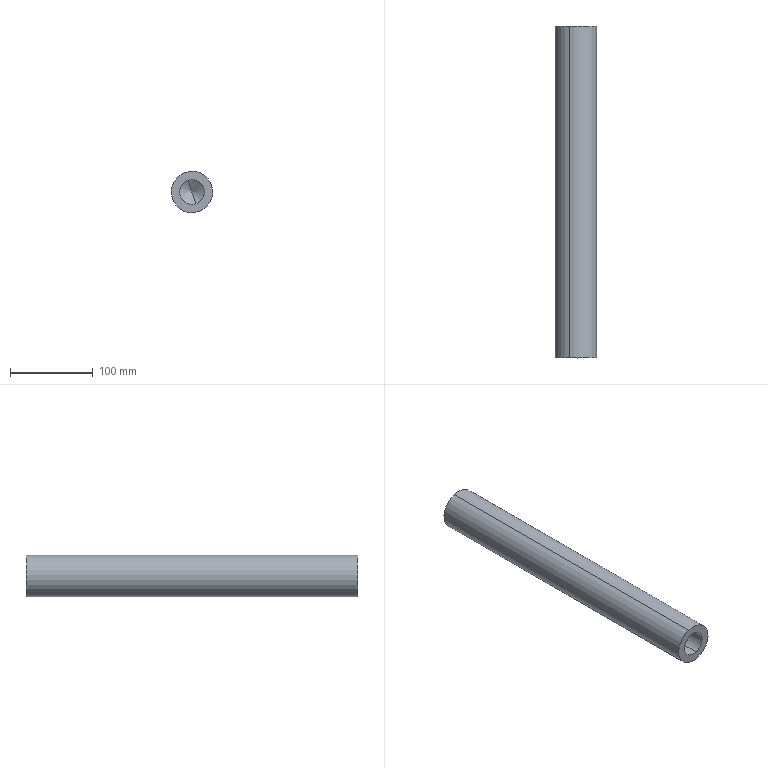Component | SolidWorks | AdjustingTieRod1-1 | 1 solid | 12 faces | box 50 x 400 x 50 mm | volume 639779 mm3 | cylinder 6 | cone 4 | plane 2 | commonest cylinder face diameters 30 x4 50 x2 | material N/A
build123d program:
from build123d import *

# Parameters (mm, degrees)
SKETCH2_R              = 25
BOSS_EXTRUDE1_DEPTH    = 400
M30_TAPPED_HOLE1_D     = 30
M30_TAPPED_HOLE1_DEPTH = 100
M30_TAPPED_HOLE1_TIP   = 9.013
M30_TAPPED_HOLE3_D     = 30
M30_TAPPED_HOLE3_DEPTH = 100
M30_TAPPED_HOLE3_TIP   = 9.013


with BuildPart() as part:
    # Sketch2 → Boss-Extrude1 (new body)
    with BuildSketch(Plane(origin=(0, 0, 0), x_dir=(1, 0, 0), z_dir=(0, 1, 0))):
        with Locations(Location((0, 0, 0), (0, 0, 270))):
            Circle(SKETCH2_R)
    extrude(amount=BOSS_EXTRUDE1_DEPTH)

    # M30 Tapped Hole1
    with Locations(Plane(origin=(0, 400, 0), x_dir=(1, 0, 0), z_dir=(0, 1, 0))):
        with Locations((0, 0)):
            Hole(M30_TAPPED_HOLE1_D / 2, depth=M30_TAPPED_HOLE1_DEPTH)
            with Locations((0, 0, -(M30_TAPPED_HOLE1_DEPTH + M30_TAPPED_HOLE1_TIP / 2))):  # 118° drill point
                Cone(0, M30_TAPPED_HOLE1_D / 2, M30_TAPPED_HOLE1_TIP, mode=Mode.SUBTRACT)

    # M30 Tapped Hole3
    with Locations(Plane(origin=(0, 0, 0), x_dir=(-1, 0, 0), z_dir=(0, -1, 0))):
        with Locations((0, 0)):
            Hole(M30_TAPPED_HOLE3_D / 2, depth=M30_TAPPED_HOLE3_DEPTH)
            with Locations((0, 0, -(M30_TAPPED_HOLE3_DEPTH + M30_TAPPED_HOLE3_TIP / 2))):  # 118° drill point
                Cone(0, M30_TAPPED_HOLE3_D / 2, M30_TAPPED_HOLE3_TIP, mode=Mode.SUBTRACT)


solid = part.part

# Placed as in the assembly
solid = solid.moved(Location((69.344, 357.787, 17), (0, 0, 0)))
STEP:
#1=COLOUR_RGB('',0.7922,0.8196,0.9333);
#2=FILL_AREA_STYLE_COLOUR('',#1);
#3=FILL_AREA_STYLE('',(#2));
#4=SURFACE_STYLE_FILL_AREA(#3);
#5=SURFACE_SIDE_STYLE('',(#4));
#6=SURFACE_STYLE_USAGE(.BOTH.,#5);
#7=PRESENTATION_STYLE_ASSIGNMENT((#6));
#8=CARTESIAN_POINT('',(2.547,18.023,1.231));
#9=VERTEX_POINT('',#8);
#10=CARTESIAN_POINT('',(2.913,18.023,0.1078));
#11=VERTEX_POINT('',#10);
#12=CARTESIAN_POINT('',(2.73,18.023,0.6693));
#13=DIRECTION('',(-0.,-1.,-0.));
#14=DIRECTION('',(0.3098,0.,-0.9508));
#15=AXIS2_PLACEMENT_3D('',#12,#13,#14);
#16=CIRCLE('',#15,0.5906);
#17=EDGE_CURVE('',#9,#11,#16,.T.);
#18=ORIENTED_EDGE('',*,*,#17,.F.);
#19=CARTESIAN_POINT('',(2.547,14.086,1.231));
#20=VERTEX_POINT('',#19);
#21=CARTESIAN_POINT('',(2.547,14.086,1.231));
#22=DIRECTION('',(-0.,-1.,-0.));
#23=VECTOR('',#22,39.37);
#24=LINE('',#21,#23);
#25=EDGE_CURVE('',#9,#20,#24,.T.);
#26=ORIENTED_EDGE('',*,*,#25,.T.);
#27=CARTESIAN_POINT('',(2.913,14.086,0.1078));
#28=VERTEX_POINT('',#27);
#29=CARTESIAN_POINT('',(2.73,14.086,0.6693));
#30=DIRECTION('',(-0.,-1.,-0.));
#31=DIRECTION('',(0.3098,0.,-0.9508));
#32=AXIS2_PLACEMENT_3D('',#29,#30,#31);
#33=CIRCLE('',#32,0.5906);
#34=EDGE_CURVE('',#20,#28,#33,.T.);
#35=ORIENTED_EDGE('',*,*,#34,.T.);
#36=CARTESIAN_POINT('',(2.913,14.086,0.1078));
#37=DIRECTION('',(-0.,-1.,-0.));
#38=VECTOR('',#37,39.37);
#39=LINE('',#36,#38);
#40=EDGE_CURVE('',#11,#28,#39,.T.);
#41=ORIENTED_EDGE('',*,*,#40,.F.);
#42=EDGE_LOOP('',(#18,#26,#35,#41));
#43=FACE_OUTER_BOUND('',#42,.T.);
#44=CARTESIAN_POINT('',(2.73,14.086,0.6693));
#45=DIRECTION('',(-0.,-1.,-0.));
#46=DIRECTION('',(0.3098,0.,-0.9508));
#47=AXIS2_PLACEMENT_3D('',#44,#45,#46);
#48=CYLINDRICAL_SURFACE('',#47,0.5906);
#49=ADVANCED_FACE('',(#43),#48,.F.);
#50=CARTESIAN_POINT('',(2.73,18.378,0.6693));
#51=VERTEX_POINT('',#50);
#52=CARTESIAN_POINT('',(2.913,18.023,0.1078));
#53=DIRECTION('',(0.2656,-0.515,-0.815));
#54=VECTOR('',#53,39.37);
#55=LINE('',#52,#54);
#56=EDGE_CURVE('',#51,#11,#55,.T.);
#57=ORIENTED_EDGE('',*,*,#56,.F.);
#58=CARTESIAN_POINT('',(2.547,18.023,1.231));
#59=DIRECTION('',(-0.2656,-0.515,0.815));
#60=VECTOR('',#59,39.37);
#61=LINE('',#58,#60);
#62=EDGE_CURVE('',#51,#9,#61,.T.);
#63=ORIENTED_EDGE('',*,*,#62,.T.);
#64=ORIENTED_EDGE('',*,*,#17,.T.);
#65=EDGE_LOOP('',(#57,#63,#64));
#66=FACE_OUTER_BOUND('',#65,.T.);
#67=CARTESIAN_POINT('',(2.73,18.023,0.6693));
#68=DIRECTION('',(-0.,-1.,-0.));
#69=DIRECTION('',(0.3098,0.,-0.9508));
#70=AXIS2_PLACEMENT_3D('',#67,#68,#69);
#71=CONICAL_SURFACE('',#70,0.5906,1.03);
#72=ADVANCED_FACE('',(#66),#71,.F.);
#73=CARTESIAN_POINT('',(2.913,25.897,0.1078));
#74=VERTEX_POINT('',#73);
#75=CARTESIAN_POINT('',(2.547,25.897,1.231));
#76=VERTEX_POINT('',#75);
#77=CARTESIAN_POINT('',(2.73,25.897,0.6693));
#78=DIRECTION('',(0.,1.,0.));
#79=DIRECTION('',(-0.3098,0.,0.9508));
#80=AXIS2_PLACEMENT_3D('',#77,#78,#79);
#81=CIRCLE('',#80,0.5906);
#82=EDGE_CURVE('',#74,#76,#81,.T.);
#83=ORIENTED_EDGE('',*,*,#82,.F.);
#84=CARTESIAN_POINT('',(2.913,29.834,0.1078));
#85=VERTEX_POINT('',#84);
#86=CARTESIAN_POINT('',(2.913,29.834,0.1078));
#87=DIRECTION('',(0.,1.,0.));
#88=VECTOR('',#87,39.37);
#89=LINE('',#86,#88);
#90=EDGE_CURVE('',#74,#85,#89,.T.);
#91=ORIENTED_EDGE('',*,*,#90,.T.);
#92=CARTESIAN_POINT('',(2.547,29.834,1.231));
#93=VERTEX_POINT('',#92);
#94=CARTESIAN_POINT('',(2.73,29.834,0.6693));
#95=DIRECTION('',(0.,1.,0.));
#96=DIRECTION('',(-0.3098,0.,0.9508));
#97=AXIS2_PLACEMENT_3D('',#94,#95,#96);
#98=CIRCLE('',#97,0.5906);
#99=EDGE_CURVE('',#85,#93,#98,.T.);
#100=ORIENTED_EDGE('',*,*,#99,.T.);
#101=CARTESIAN_POINT('',(2.547,29.834,1.231));
#102=DIRECTION('',(0.,1.,0.));
#103=VECTOR('',#102,39.37);
#104=LINE('',#101,#103);
#105=EDGE_CURVE('',#76,#93,#104,.T.);
#106=ORIENTED_EDGE('',*,*,#105,.F.);
#107=EDGE_LOOP('',(#83,#91,#100,#106));
#108=FACE_OUTER_BOUND('',#107,.T.);
#109=CARTESIAN_POINT('',(2.73,29.834,0.6693));
#110=DIRECTION('',(0.,1.,0.));
#111=DIRECTION('',(-0.3098,0.,0.9508));
#112=AXIS2_PLACEMENT_3D('',#109,#110,#111);
#113=CYLINDRICAL_SURFACE('',#112,0.5906);
#114=ADVANCED_FACE('',(#108),#113,.F.);
#115=CARTESIAN_POINT('',(2.73,25.542,0.6693));
#116=VERTEX_POINT('',#115);
#117=CARTESIAN_POINT('',(2.547,25.897,1.231));
#118=DIRECTION('',(-0.2656,0.515,0.815));
#119=VECTOR('',#118,39.37);
#120=LINE('',#117,#119);
#121=EDGE_CURVE('',#116,#76,#120,.T.);
#122=ORIENTED_EDGE('',*,*,#121,.F.);
#123=CARTESIAN_POINT('',(2.913,25.897,0.1078));
#124=DIRECTION('',(0.2656,0.515,-0.815));
#125=VECTOR('',#124,39.37);
#126=LINE('',#123,#125);
#127=EDGE_CURVE('',#116,#74,#126,.T.);
#128=ORIENTED_EDGE('',*,*,#127,.T.);
#129=ORIENTED_EDGE('',*,*,#82,.T.);
#130=EDGE_LOOP('',(#122,#128,#129));
#131=FACE_OUTER_BOUND('',#130,.T.);
#132=CARTESIAN_POINT('',(2.73,25.897,0.6693));
#133=DIRECTION('',(0.,1.,0.));
#134=DIRECTION('',(-0.3098,0.,0.9508));
#135=AXIS2_PLACEMENT_3D('',#132,#133,#134);
#136=CONICAL_SURFACE('',#135,0.5906,1.03);
#137=ADVANCED_FACE('',(#131),#136,.F.);
#138=CARTESIAN_POINT('',(2.425,29.834,1.605));
#139=VERTEX_POINT('',#138);
#140=CARTESIAN_POINT('',(3.035,29.834,-0.2665));
#141=VERTEX_POINT('',#140);
#142=CARTESIAN_POINT('',(2.73,29.834,0.6693));
#143=DIRECTION('',(0.,1.,0.));
#144=DIRECTION('',(-0.3098,0.,0.9508));
#145=AXIS2_PLACEMENT_3D('',#142,#143,#144);
#146=CIRCLE('',#145,0.9843);
#147=EDGE_CURVE('',#139,#141,#146,.T.);
#148=ORIENTED_EDGE('',*,*,#147,.F.);
#149=CARTESIAN_POINT('',(2.425,14.086,1.605));
#150=VERTEX_POINT('',#149);
#151=CARTESIAN_POINT('',(2.425,29.834,1.605));
#152=DIRECTION('',(-0.,-1.,-0.));
#153=VECTOR('',#152,39.37);
#154=LINE('',#151,#153);
#155=EDGE_CURVE('',#139,#150,#154,.T.);
#156=ORIENTED_EDGE('',*,*,#155,.T.);
#157=CARTESIAN_POINT('',(3.035,14.086,-0.2665));
#158=VERTEX_POINT('',#157);
#159=CARTESIAN_POINT('',(2.73,14.086,0.6693));
#160=DIRECTION('',(0.,1.,0.));
#161=DIRECTION('',(-0.3098,0.,0.9508));
#162=AXIS2_PLACEMENT_3D('',#159,#160,#161);
#163=CIRCLE('',#162,0.9843);
#164=EDGE_CURVE('',#150,#158,#163,.T.);
#165=ORIENTED_EDGE('',*,*,#164,.T.);
#166=CARTESIAN_POINT('',(3.035,29.834,-0.2665));
#167=DIRECTION('',(-0.,-1.,-0.));
#168=VECTOR('',#167,39.37);
#169=LINE('',#166,#168);
#170=EDGE_CURVE('',#141,#158,#169,.T.);
#171=ORIENTED_EDGE('',*,*,#170,.F.);
#172=EDGE_LOOP('',(#148,#156,#165,#171));
#173=FACE_OUTER_BOUND('',#172,.T.);
#174=CARTESIAN_POINT('',(2.73,29.834,0.6693));
#175=DIRECTION('',(-0.,-1.,-0.));
#176=DIRECTION('',(0.3098,0.,-0.9508));
#177=AXIS2_PLACEMENT_3D('',#174,#175,#176);
#178=CYLINDRICAL_SURFACE('',#177,0.9843);
#179=ADVANCED_FACE('',(#173),#178,.T.);
#180=ORIENTED_EDGE('',*,*,#155,.F.);
#181=CARTESIAN_POINT('',(2.73,29.834,0.6693));
#182=DIRECTION('',(0.,1.,0.));
#183=DIRECTION('',(-0.3098,0.,0.9508));
#184=AXIS2_PLACEMENT_3D('',#181,#182,#183);
#185=CIRCLE('',#184,0.9843);
#186=EDGE_CURVE('',#141,#139,#185,.T.);
#187=ORIENTED_EDGE('',*,*,#186,.F.);
#188=ORIENTED_EDGE('',*,*,#170,.T.);
#189=CARTESIAN_POINT('',(2.73,14.086,0.6693));
#190=DIRECTION('',(0.,1.,0.));
#191=DIRECTION('',(-0.3098,0.,0.9508));
#192=AXIS2_PLACEMENT_3D('',#189,#190,#191);
#193=CIRCLE('',#192,0.9843);
#194=EDGE_CURVE('',#158,#150,#193,.T.);
#195=ORIENTED_EDGE('',*,*,#194,.T.);
#196=EDGE_LOOP('',(#180,#187,#188,#195));
#197=FACE_OUTER_BOUND('',#196,.T.);
#198=CARTESIAN_POINT('',(2.73,29.834,0.6693));
#199=DIRECTION('',(-0.,-1.,-0.));
#200=DIRECTION('',(0.3098,0.,-0.9508));
#201=AXIS2_PLACEMENT_3D('',#198,#199,#200);
#202=CYLINDRICAL_SURFACE('',#201,0.9843);
#203=ADVANCED_FACE('',(#197),#202,.T.);
#204=CARTESIAN_POINT('',(2.73,29.834,0.6693));
#205=DIRECTION('',(0.,1.,0.));
#206=DIRECTION('',(-0.3098,0.,0.9508));
#207=AXIS2_PLACEMENT_3D('',#204,#205,#206);
#208=CIRCLE('',#207,0.5906);
#209=EDGE_CURVE('',#93,#85,#208,.T.);
#210=ORIENTED_EDGE('',*,*,#209,.F.);
#211=ORIENTED_EDGE('',*,*,#99,.F.);
#212=EDGE_LOOP('',(#210,#211));
#213=FACE_BOUND('',#212,.T.);
#214=ORIENTED_EDGE('',*,*,#186,.T.);
#215=ORIENTED_EDGE('',*,*,#147,.T.);
#216=EDGE_LOOP('',(#214,#215));
#217=FACE_OUTER_BOUND('',#216,.T.);
#218=CARTESIAN_POINT('',(2.73,29.834,0.6693));
#219=DIRECTION('',(0.,1.,0.));
#220=DIRECTION('',(-0.3098,0.,0.9508));
#221=AXIS2_PLACEMENT_3D('',#218,#219,#220);
#222=PLANE('',#221);
#223=ADVANCED_FACE('',(#213,#217),#222,.T.);
#224=CARTESIAN_POINT('',(2.73,14.086,0.6693));
#225=DIRECTION('',(-0.,-1.,-0.));
#226=DIRECTION('',(0.3098,0.,-0.9508));
#227=AXIS2_PLACEMENT_3D('',#224,#225,#226);
#228=CIRCLE('',#227,0.5906);
#229=EDGE_CURVE('',#28,#20,#228,.T.);
#230=ORIENTED_EDGE('',*,*,#229,.F.);
#231=ORIENTED_EDGE('',*,*,#34,.F.);
#232=EDGE_LOOP('',(#230,#231));
#233=FACE_BOUND('',#232,.T.);
#234=ORIENTED_EDGE('',*,*,#194,.F.);
#235=ORIENTED_EDGE('',*,*,#164,.F.);
#236=EDGE_LOOP('',(#234,#235));
#237=FACE_OUTER_BOUND('',#236,.T.);
#238=CARTESIAN_POINT('',(2.73,14.086,0.6693));
#239=DIRECTION('',(0.,1.,0.));
#240=DIRECTION('',(-0.3098,0.,0.9508));
#241=AXIS2_PLACEMENT_3D('',#238,#239,#240);
#242=PLANE('',#241);
#243=ADVANCED_FACE('',(#233,#237),#242,.F.);
#244=ORIENTED_EDGE('',*,*,#127,.F.);
#245=ORIENTED_EDGE('',*,*,#121,.T.);
#246=CARTESIAN_POINT('',(2.73,25.897,0.6693));
#247=DIRECTION('',(0.,1.,0.));
#248=DIRECTION('',(-0.3098,0.,0.9508));
#249=AXIS2_PLACEMENT_3D('',#246,#247,#248);
#250=CIRCLE('',#249,0.5906);
#251=EDGE_CURVE('',#76,#74,#250,.T.);
#252=ORIENTED_EDGE('',*,*,#251,.T.);
#253=EDGE_LOOP('',(#244,#245,#252));
#254=FACE_OUTER_BOUND('',#253,.T.);
#255=CARTESIAN_POINT('',(2.73,25.897,0.6693));
#256=DIRECTION('',(0.,1.,0.));
#257=DIRECTION('',(-0.3098,0.,0.9508));
#258=AXIS2_PLACEMENT_3D('',#255,#256,#257);
#259=CONICAL_SURFACE('',#258,0.5906,1.03);
#260=ADVANCED_FACE('',(#254),#259,.F.);
#261=ORIENTED_EDGE('',*,*,#90,.F.);
#262=ORIENTED_EDGE('',*,*,#251,.F.);
#263=ORIENTED_EDGE('',*,*,#105,.T.);
#264=ORIENTED_EDGE('',*,*,#209,.T.);
#265=EDGE_LOOP('',(#261,#262,#263,#264));
#266=FACE_OUTER_BOUND('',#265,.T.);
#267=CARTESIAN_POINT('',(2.73,29.834,0.6693));
#268=DIRECTION('',(0.,1.,0.));
#269=DIRECTION('',(-0.3098,0.,0.9508));
#270=AXIS2_PLACEMENT_3D('',#267,#268,#269);
#271=CYLINDRICAL_SURFACE('',#270,0.5906);
#272=ADVANCED_FACE('',(#266),#271,.F.);
#273=ORIENTED_EDGE('',*,*,#62,.F.);
#274=ORIENTED_EDGE('',*,*,#56,.T.);
#275=CARTESIAN_POINT('',(2.73,18.023,0.6693));
#276=DIRECTION('',(-0.,-1.,-0.));
#277=DIRECTION('',(0.3098,0.,-0.9508));
#278=AXIS2_PLACEMENT_3D('',#275,#276,#277);
#279=CIRCLE('',#278,0.5906);
#280=EDGE_CURVE('',#11,#9,#279,.T.);
#281=ORIENTED_EDGE('',*,*,#280,.T.);
#282=EDGE_LOOP('',(#273,#274,#281));
#283=FACE_OUTER_BOUND('',#282,.T.);
#284=CARTESIAN_POINT('',(2.73,18.023,0.6693));
#285=DIRECTION('',(-0.,-1.,-0.));
#286=DIRECTION('',(0.3098,0.,-0.9508));
#287=AXIS2_PLACEMENT_3D('',#284,#285,#286);
#288=CONICAL_SURFACE('',#287,0.5906,1.03);
#289=ADVANCED_FACE('',(#283),#288,.F.);
#290=ORIENTED_EDGE('',*,*,#25,.F.);
#291=ORIENTED_EDGE('',*,*,#280,.F.);
#292=ORIENTED_EDGE('',*,*,#40,.T.);
#293=ORIENTED_EDGE('',*,*,#229,.T.);
#294=EDGE_LOOP('',(#290,#291,#292,#293));
#295=FACE_OUTER_BOUND('',#294,.T.);
#296=CARTESIAN_POINT('',(2.73,14.086,0.6693));
#297=DIRECTION('',(-0.,-1.,-0.));
#298=DIRECTION('',(0.3098,0.,-0.9508));
#299=AXIS2_PLACEMENT_3D('',#296,#297,#298);
#300=CYLINDRICAL_SURFACE('',#299,0.5906);
#301=ADVANCED_FACE('',(#295),#300,.F.);
#302=CLOSED_SHELL('',(#49,#72,#114,#137,#179,#203,#223,#243,#260,#272,#289,#301));
#303=MANIFOLD_SOLID_BREP('',#302);
#304=STYLED_ITEM('',(#7),#303);
#305=PRESENTATION_LAYER_ASSIGNMENT('','',(#304));
#306=CARTESIAN_POINT('',(0.,0.,0.));
#307=DIRECTION('',(0.,0.,1.));
#308=DIRECTION('',(1.,0.,0.));
#309=AXIS2_PLACEMENT_3D('',#306,#307,#308);
#310=(LENGTH_UNIT()NAMED_UNIT(*)SI_UNIT($,.METRE.));
#311=LENGTH_MEASURE_WITH_UNIT(LENGTH_MEASURE(0.0254),#310);
#312=DIMENSIONAL_EXPONENTS(1.,0.,0.,0.,0.,0.,0.);
#313=(CONVERSION_BASED_UNIT('',#311)LENGTH_UNIT()NAMED_UNIT(#312));
#314=UNCERTAINTY_MEASURE_WITH_UNIT(LENGTH_MEASURE(0.00001),#313,'','');
#315=(NAMED_UNIT(*)PLANE_ANGLE_UNIT()SI_UNIT($,.RADIAN.));
#316=(NAMED_UNIT(*)SI_UNIT($,.STERADIAN.)SOLID_ANGLE_UNIT());
#317=(GEOMETRIC_REPRESENTATION_CONTEXT(3)GLOBAL_UNCERTAINTY_ASSIGNED_CONTEXT((#314))GLOBAL_UNIT_ASSIGNED_CONTEXT((#313,#315,#316))REPRESENTATION_CONTEXT('',''));
#318=ADVANCED_BREP_SHAPE_REPRESENTATION('',(#303,#309),#317);
#319=(LENGTH_UNIT()NAMED_UNIT(*)SI_UNIT($,.METRE.));
#320=LENGTH_MEASURE_WITH_UNIT(LENGTH_MEASURE(0.0254),#319);
#321=DIMENSIONAL_EXPONENTS(1.,0.,0.,0.,0.,0.,0.);
#322=(CONVERSION_BASED_UNIT('',#320)LENGTH_UNIT()NAMED_UNIT(#321));
#323=UNCERTAINTY_MEASURE_WITH_UNIT(LENGTH_MEASURE(0.00001),#322,'','');
#324=(NAMED_UNIT(*)PLANE_ANGLE_UNIT()SI_UNIT($,.RADIAN.));
#325=(NAMED_UNIT(*)SI_UNIT($,.STERADIAN.)SOLID_ANGLE_UNIT());
#326=(GEOMETRIC_REPRESENTATION_CONTEXT(3)GLOBAL_UNCERTAINTY_ASSIGNED_CONTEXT((#323))GLOBAL_UNIT_ASSIGNED_CONTEXT((#322,#324,#325))REPRESENTATION_CONTEXT('',''));
#327=MECHANICAL_DESIGN_GEOMETRIC_PRESENTATION_REPRESENTATION('',(#304),#326);